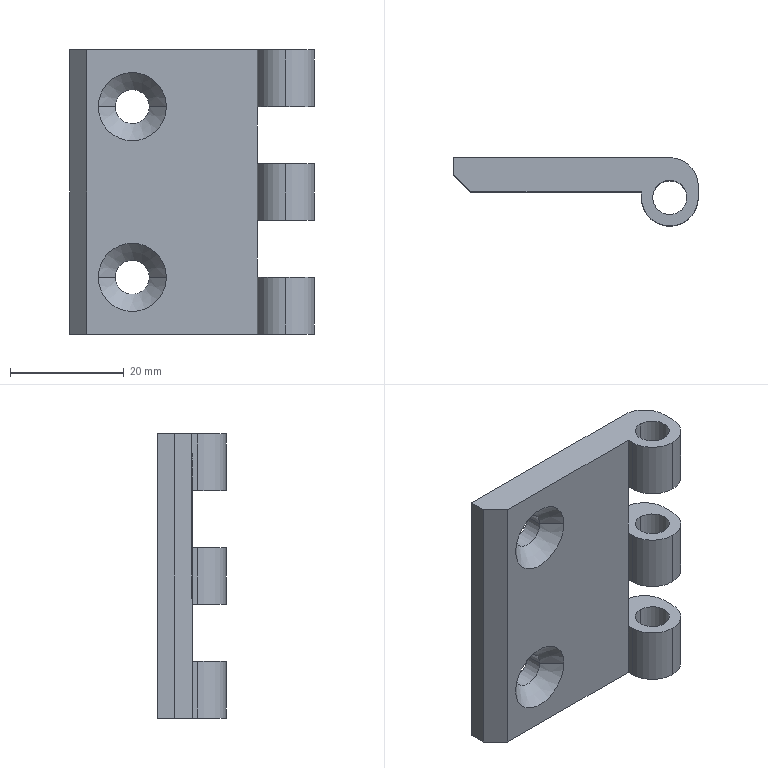Component | SolidWorks | OuterDoorHingeAssembly1-1_OuterDoorHinge3-1 | 1 solid | 41 faces | volume 11378 mm3 | cylinder 19 | plane 18 | cone 4 | commonest cylinder face diameters 6 x10 10 x9